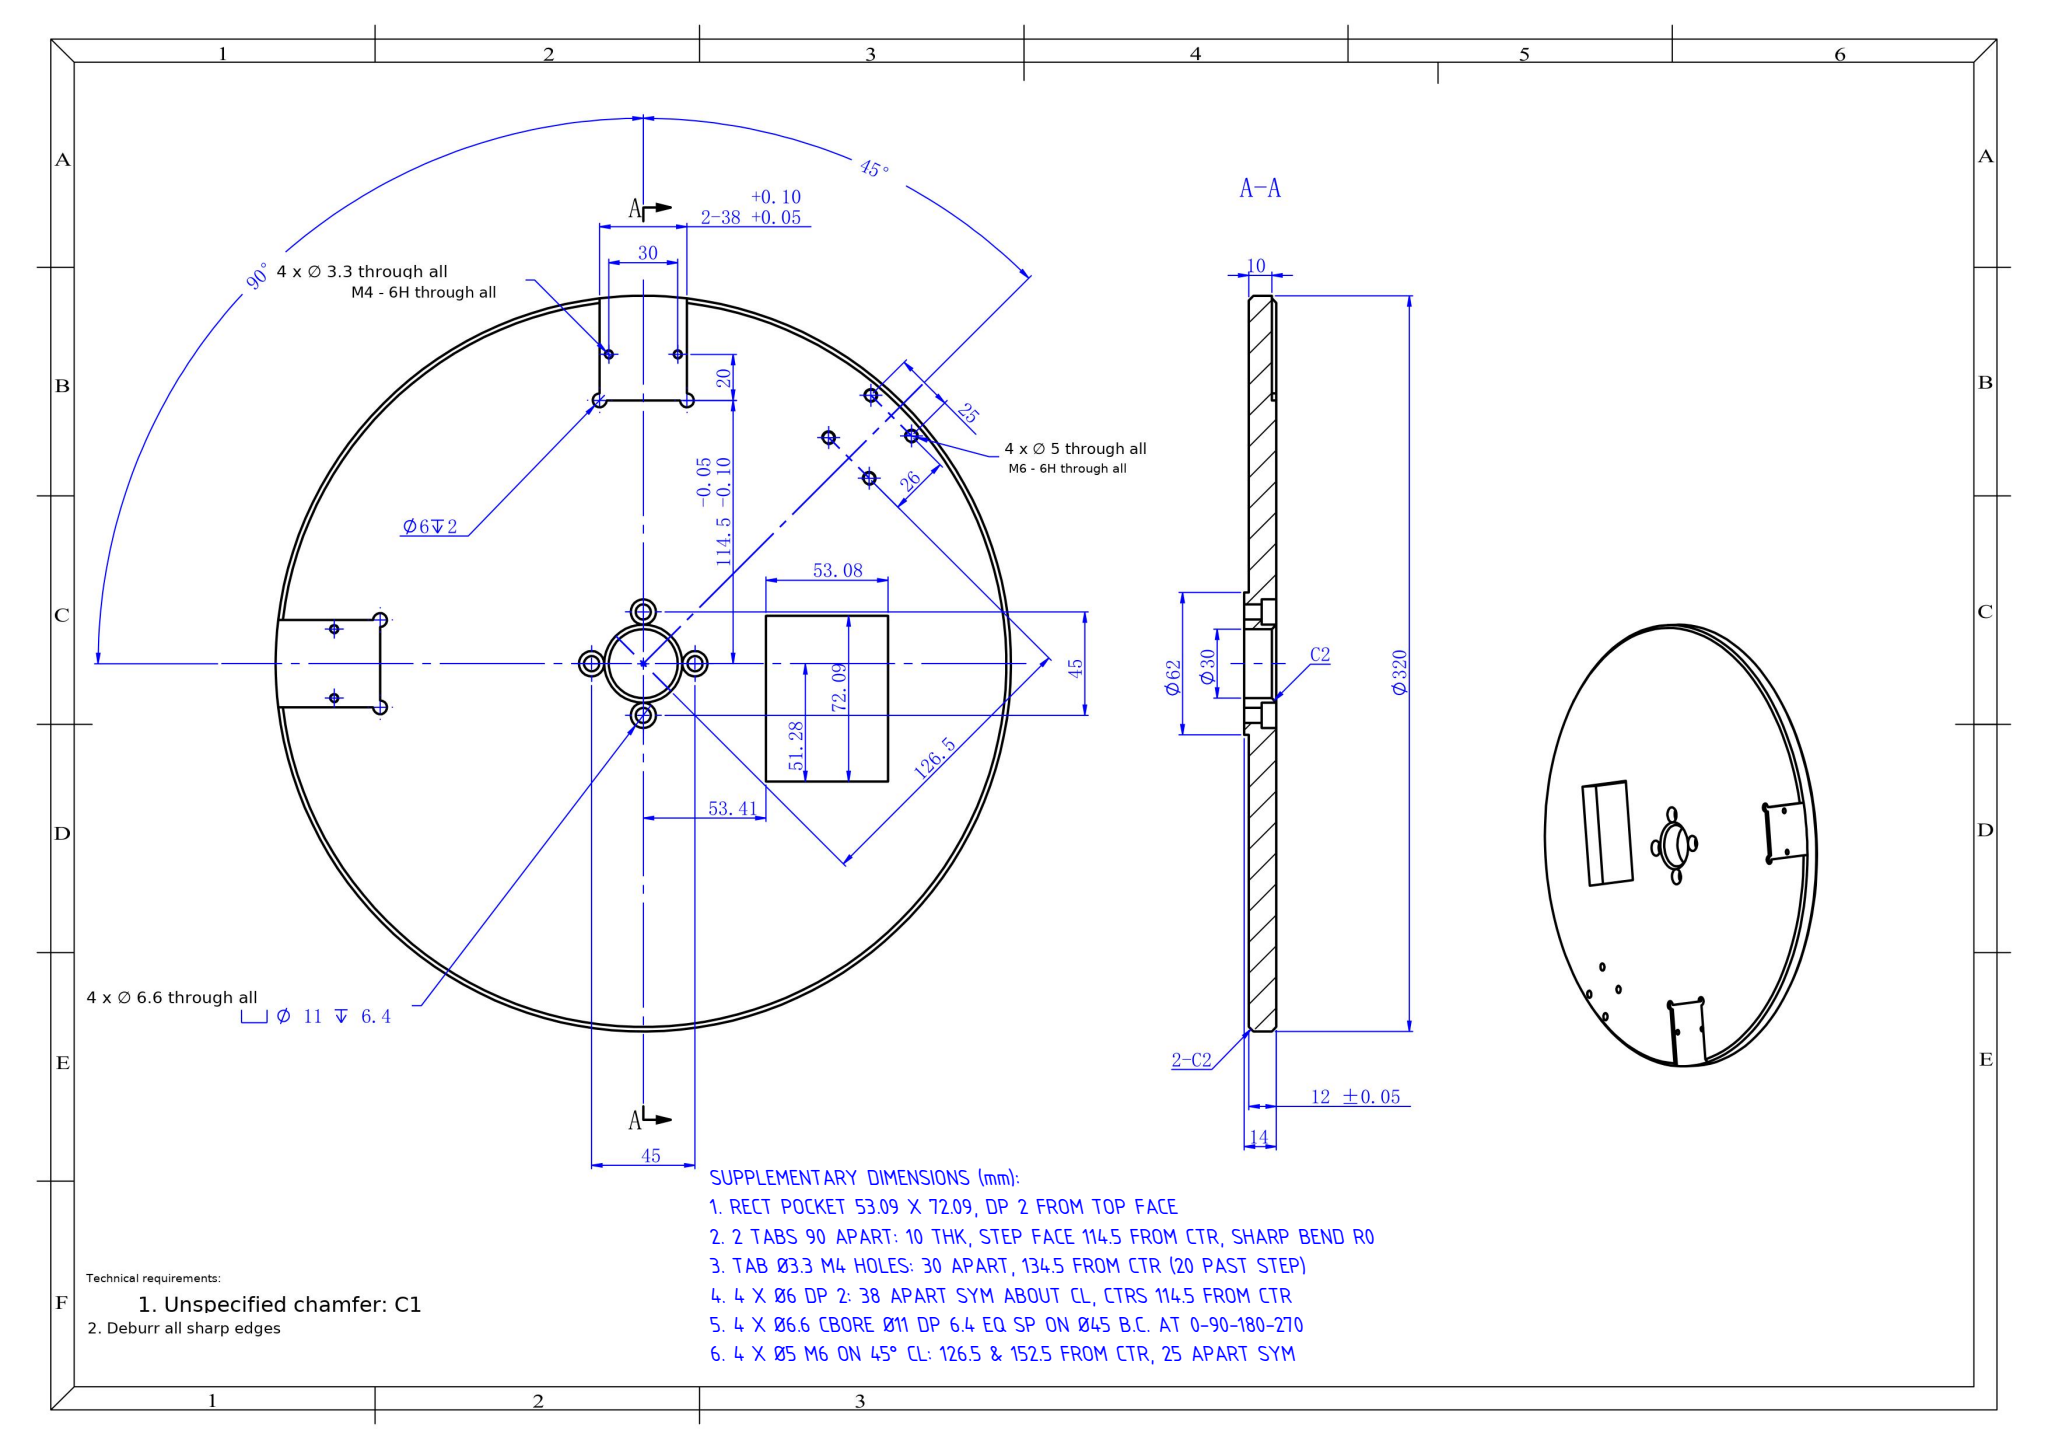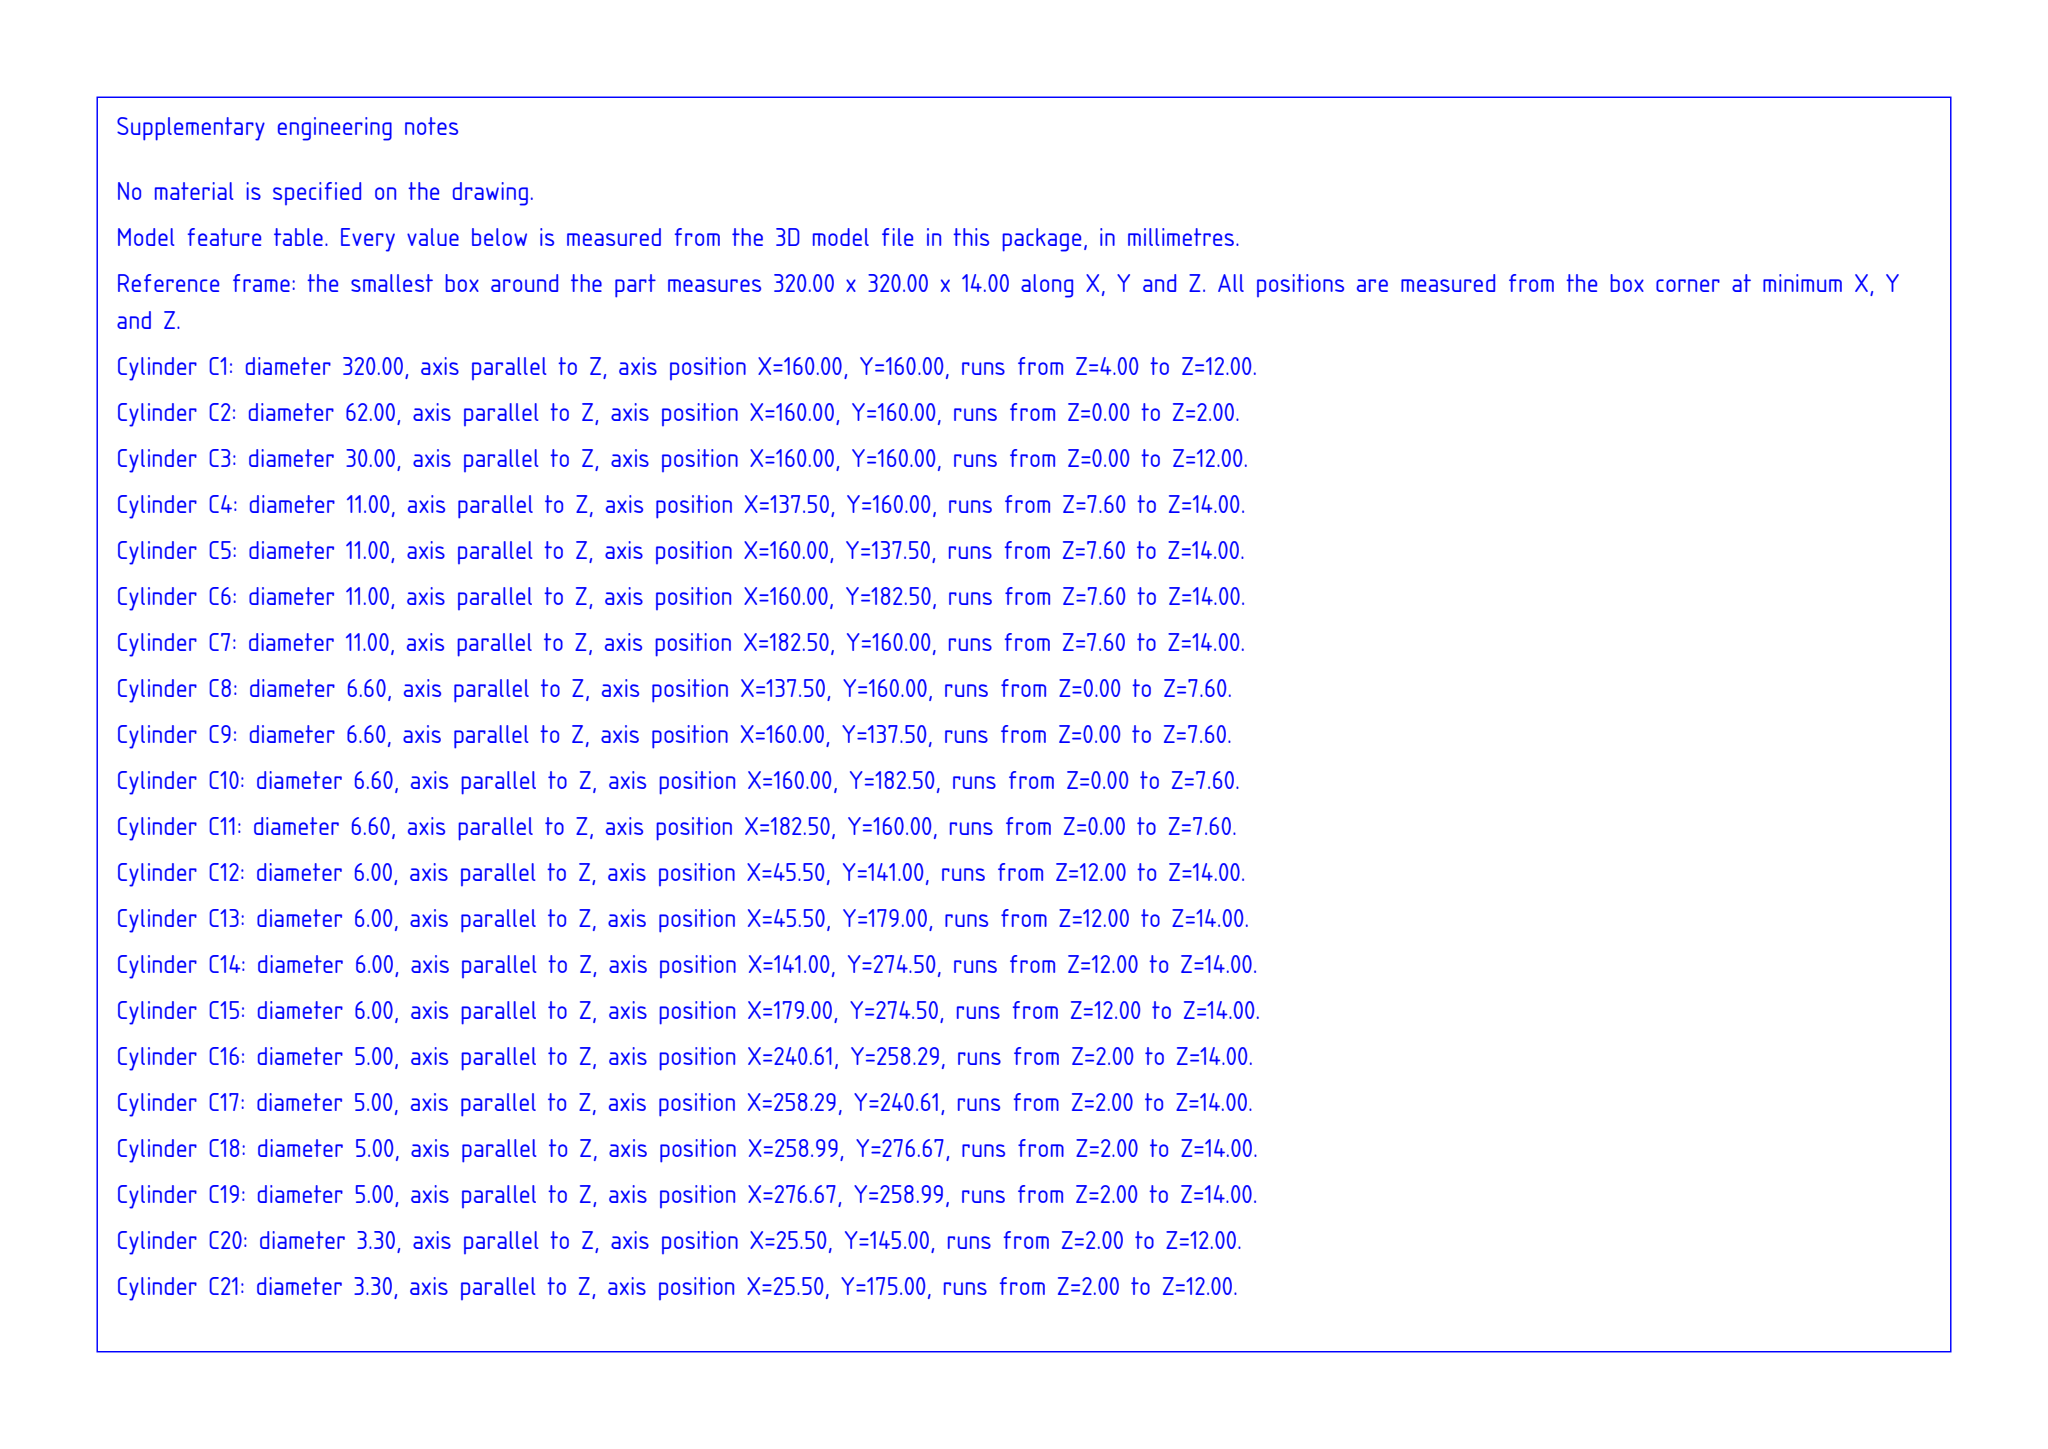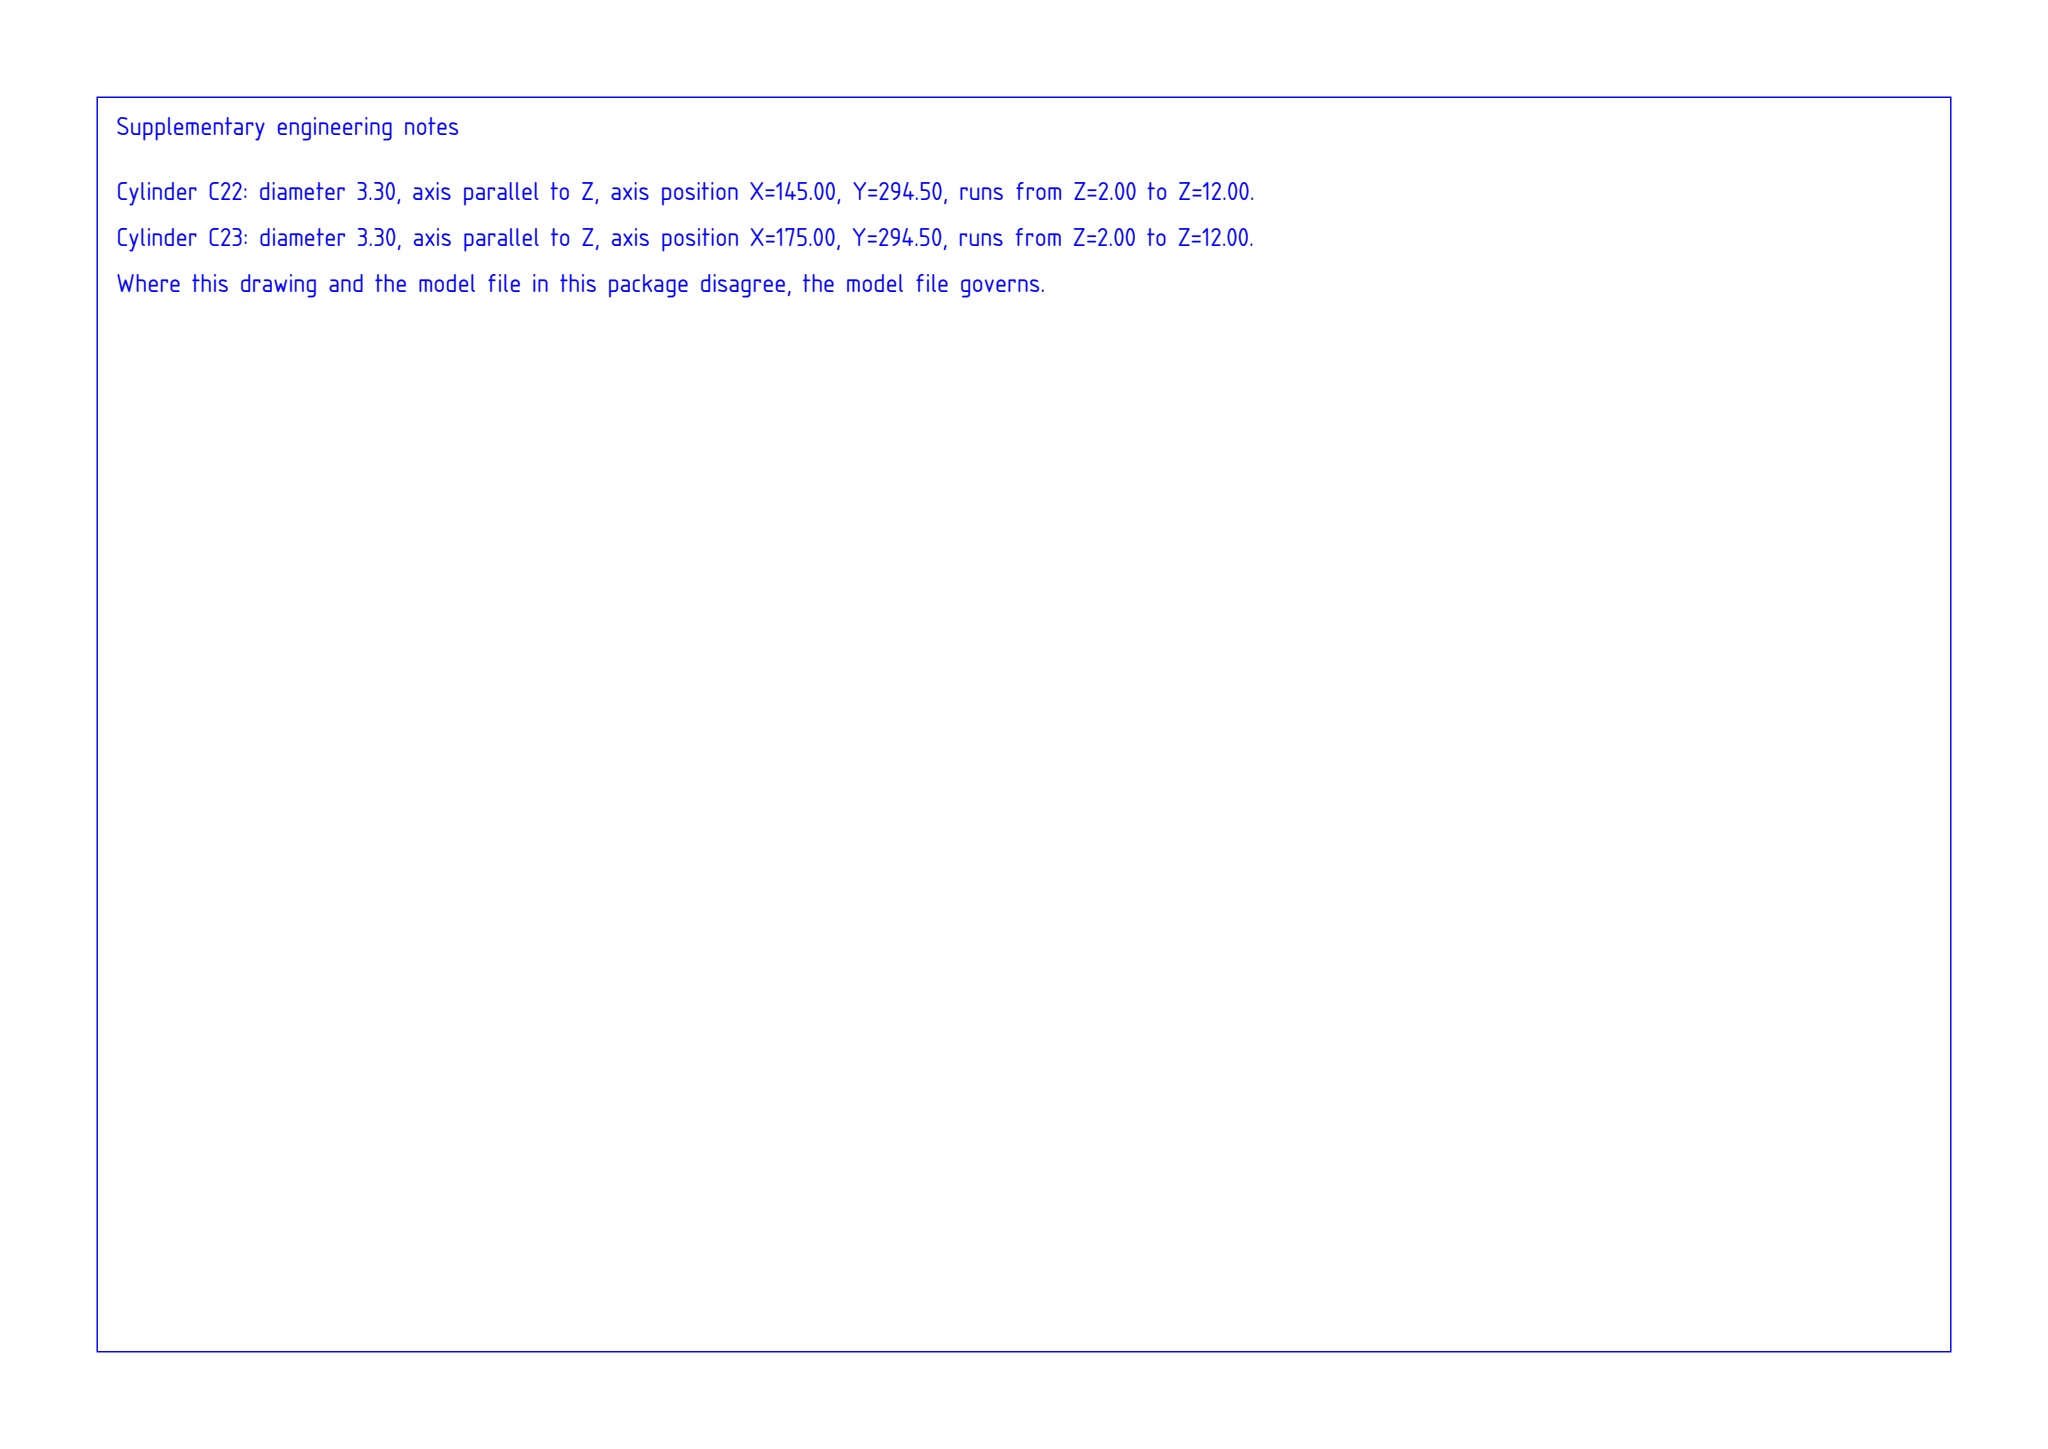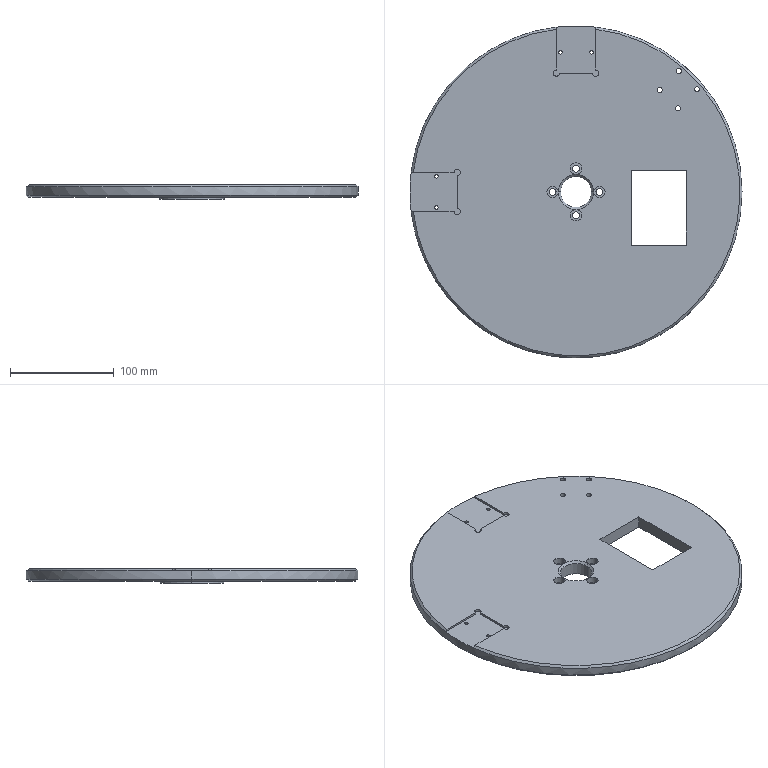Part | SolidWorks | mm | 1 solid | 70 faces | box 320 x 320 x 14 mm | volume 899482 mm3 | cylinder 45 | plane 19 | cone 6 | commonest cylinder face diameters 5 x8 11 x8 6.6 x8 3.3 x8 6 x7 62 x2 30 x2 320 x2